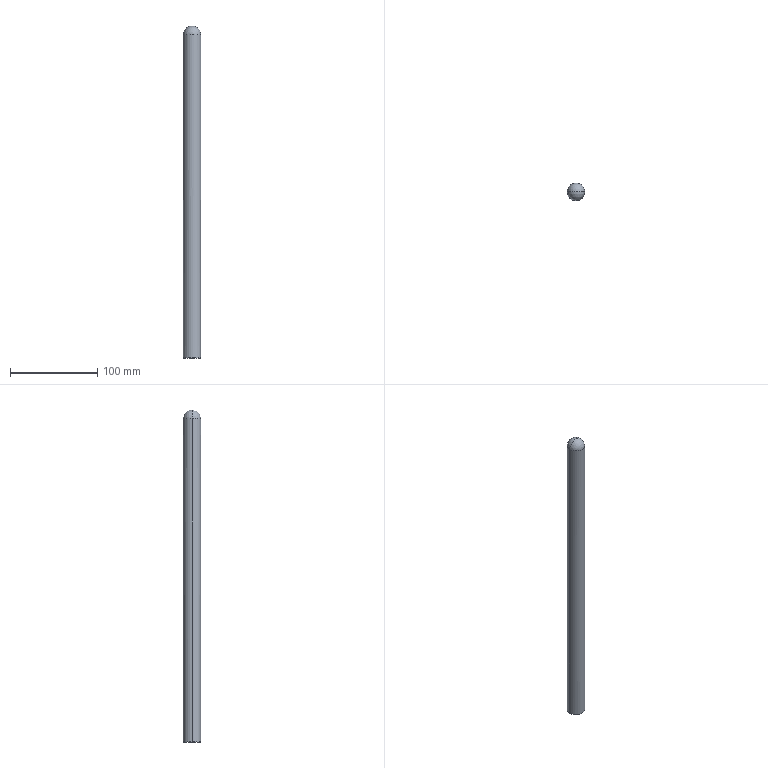Component | SolidWorks | 002MaterialPickingModuleB-1_J-003-2 | 1 solid | 11 faces | box 20 x 20 x 380 mm | volume 117584 mm3 | cone 4 | cylinder 4 | sphere 2 | plane 1 | commonest cylinder face diameters 6.8 x2 20 x2 | material 45
build123d program:
from build123d import *

# Parameters (mm, degrees)
SKETCH1_R             = 10
BOSS_EXTRUDE1_DEPTH   = 380
M8_TAPPED_HOLE1_D     = 6.8
M8_TAPPED_HOLE1_DEPTH = 19.75
M8_TAPPED_HOLE1_TIP   = 2.043
FILLET1_R             = 10
CHAMFER1_SIZE         = 0.5


with BuildPart() as part:
    # Sketch1 → Boss-Extrude1 (new body)
    with BuildSketch(Plane.XY):
        Circle(SKETCH1_R)
    extrude(amount=BOSS_EXTRUDE1_DEPTH)

    # M8 Tapped Hole1
    with Locations(Plane(origin=(0, 0, 0), x_dir=(-1, 0, 0), z_dir=(0, 0, -1))):
        with Locations((0, 0)):
            Hole(M8_TAPPED_HOLE1_D / 2, depth=M8_TAPPED_HOLE1_DEPTH)
            with Locations((0, 0, -(M8_TAPPED_HOLE1_DEPTH + M8_TAPPED_HOLE1_TIP / 2))):  # 118° drill point
                Cone(0, M8_TAPPED_HOLE1_D / 2, M8_TAPPED_HOLE1_TIP, mode=Mode.SUBTRACT)

    # Fillet1
    fillet1_edges = [part.edges().sort_by_distance(p)[0] for p in [
        (-10, 0, 380),
    ]]
    fillet(fillet1_edges, radius=FILLET1_R)

    # Chamfer1
    chamfer1_edges = [part.edges().sort_by_distance(p)[0] for p in [
        (-10, 0, 0),
    ]]
    chamfer(chamfer1_edges, length=CHAMFER1_SIZE)


solid = part.part

# Placed as in the assembly
solid = solid.moved(Location((70.325, 123.019, 113.231), (0, 0, 0)))
STEP:
#1=CARTESIAN_POINT('',(2.395,4.843,4.458));
#2=VERTEX_POINT('',#1);
#3=CARTESIAN_POINT('',(3.143,4.843,4.458));
#4=VERTEX_POINT('',#3);
#5=CARTESIAN_POINT('',(2.769,4.843,4.458));
#6=DIRECTION('',(0.,0.,-1.));
#7=DIRECTION('',(1.,0.,0.));
#8=AXIS2_PLACEMENT_3D('',#5,#6,#7);
#9=CIRCLE('',#8,0.374);
#10=EDGE_CURVE('',#2,#4,#9,.T.);
#11=ORIENTED_EDGE('',*,*,#10,.F.);
#12=CARTESIAN_POINT('',(2.375,4.843,4.478));
#13=VERTEX_POINT('',#12);
#14=CARTESIAN_POINT('',(2.375,4.843,4.478));
#15=DIRECTION('',(-0.7071,0.,0.7071));
#16=VECTOR('',#15,39.37);
#17=LINE('',#14,#16);
#18=EDGE_CURVE('',#2,#13,#17,.T.);
#19=ORIENTED_EDGE('',*,*,#18,.T.);
#20=CARTESIAN_POINT('',(3.162,4.843,4.478));
#21=VERTEX_POINT('',#20);
#22=CARTESIAN_POINT('',(2.769,4.843,4.478));
#23=DIRECTION('',(0.,0.,1.));
#24=DIRECTION('',(1.,0.,0.));
#25=AXIS2_PLACEMENT_3D('',#22,#23,#24);
#26=CIRCLE('',#25,0.3937);
#27=EDGE_CURVE('',#21,#13,#26,.T.);
#28=ORIENTED_EDGE('',*,*,#27,.F.);
#29=CARTESIAN_POINT('',(3.162,4.843,4.478));
#30=DIRECTION('',(0.7071,0.,0.7071));
#31=VECTOR('',#30,39.37);
#32=LINE('',#29,#31);
#33=EDGE_CURVE('',#4,#21,#32,.T.);
#34=ORIENTED_EDGE('',*,*,#33,.F.);
#35=EDGE_LOOP('',(#11,#19,#28,#34));
#36=FACE_OUTER_BOUND('',#35,.T.);
#37=CARTESIAN_POINT('',(2.769,4.843,4.478));
#38=DIRECTION('',(0.,0.,1.));
#39=DIRECTION('',(1.,0.,0.));
#40=AXIS2_PLACEMENT_3D('',#37,#38,#39);
#41=CONICAL_SURFACE('',#40,0.3937,0.7854);
#42=ADVANCED_FACE('',(#36),#41,.T.);
#43=CARTESIAN_POINT('',(2.375,4.843,19.025));
#44=VERTEX_POINT('',#43);
#45=CARTESIAN_POINT('',(3.162,4.843,19.025));
#46=VERTEX_POINT('',#45);
#47=CARTESIAN_POINT('',(2.769,4.843,19.025));
#48=DIRECTION('',(0.,0.,-1.));
#49=DIRECTION('',(-1.,0.,0.));
#50=AXIS2_PLACEMENT_3D('',#47,#48,#49);
#51=CIRCLE('',#50,0.3937);
#52=EDGE_CURVE('',#44,#46,#51,.T.);
#53=ORIENTED_EDGE('',*,*,#52,.F.);
#54=CARTESIAN_POINT('',(2.769,4.843,19.419));
#55=VERTEX_POINT('',#54);
#56=CARTESIAN_POINT('',(2.769,4.843,19.025));
#57=DIRECTION('',(0.,1.,0.));
#58=DIRECTION('',(-1.,0.,0.));
#59=AXIS2_PLACEMENT_3D('',#56,#57,#58);
#60=CIRCLE('',#59,0.3937);
#61=EDGE_CURVE('',#44,#55,#60,.T.);
#62=ORIENTED_EDGE('',*,*,#61,.T.);
#63=CARTESIAN_POINT('',(2.769,4.843,19.025));
#64=DIRECTION('',(0.,-1.,0.));
#65=DIRECTION('',(0.,0.,-1.));
#66=AXIS2_PLACEMENT_3D('',#63,#64,#65);
#67=CIRCLE('',#66,0.3937);
#68=EDGE_CURVE('',#46,#55,#67,.T.);
#69=ORIENTED_EDGE('',*,*,#68,.F.);
#70=EDGE_LOOP('',(#53,#62,#69));
#71=FACE_OUTER_BOUND('',#70,.T.);
#72=CARTESIAN_POINT('',(2.769,4.843,19.025));
#73=DIRECTION('',(0.,1.,0.));
#74=DIRECTION('',(1.,0.,0.));
#75=AXIS2_PLACEMENT_3D('',#72,#73,#74);
#76=SPHERICAL_SURFACE('',#75,0.3937);
#77=ADVANCED_FACE('',(#71),#76,.T.);
#78=CARTESIAN_POINT('',(2.903,4.843,5.235));
#79=VERTEX_POINT('',#78);
#80=CARTESIAN_POINT('',(2.635,4.843,5.235));
#81=VERTEX_POINT('',#80);
#82=CARTESIAN_POINT('',(2.769,4.843,5.235));
#83=DIRECTION('',(0.,0.,-1.));
#84=DIRECTION('',(-1.,0.,0.));
#85=AXIS2_PLACEMENT_3D('',#82,#83,#84);
#86=CIRCLE('',#85,0.1339);
#87=EDGE_CURVE('',#79,#81,#86,.T.);
#88=ORIENTED_EDGE('',*,*,#87,.F.);
#89=CARTESIAN_POINT('',(2.903,4.843,4.458));
#90=VERTEX_POINT('',#89);
#91=CARTESIAN_POINT('',(2.903,4.843,4.458));
#92=DIRECTION('',(0.,0.,-1.));
#93=VECTOR('',#92,39.37);
#94=LINE('',#91,#93);
#95=EDGE_CURVE('',#79,#90,#94,.T.);
#96=ORIENTED_EDGE('',*,*,#95,.T.);
#97=CARTESIAN_POINT('',(2.635,4.843,4.458));
#98=VERTEX_POINT('',#97);
#99=CARTESIAN_POINT('',(2.769,4.843,4.458));
#100=DIRECTION('',(0.,0.,-1.));
#101=DIRECTION('',(-1.,0.,0.));
#102=AXIS2_PLACEMENT_3D('',#99,#100,#101);
#103=CIRCLE('',#102,0.1339);
#104=EDGE_CURVE('',#90,#98,#103,.T.);
#105=ORIENTED_EDGE('',*,*,#104,.T.);
#106=CARTESIAN_POINT('',(2.635,4.843,4.458));
#107=DIRECTION('',(0.,0.,-1.));
#108=VECTOR('',#107,39.37);
#109=LINE('',#106,#108);
#110=EDGE_CURVE('',#81,#98,#109,.T.);
#111=ORIENTED_EDGE('',*,*,#110,.F.);
#112=EDGE_LOOP('',(#88,#96,#105,#111));
#113=FACE_OUTER_BOUND('',#112,.T.);
#114=CARTESIAN_POINT('',(2.769,4.843,4.458));
#115=DIRECTION('',(0.,0.,-1.));
#116=DIRECTION('',(-1.,0.,0.));
#117=AXIS2_PLACEMENT_3D('',#114,#115,#116);
#118=CYLINDRICAL_SURFACE('',#117,0.1339);
#119=ADVANCED_FACE('',(#113),#118,.F.);
#120=CARTESIAN_POINT('',(2.769,4.843,5.316));
#121=VERTEX_POINT('',#120);
#122=CARTESIAN_POINT('',(2.635,4.843,5.235));
#123=DIRECTION('',(-0.8572,0.,-0.515));
#124=VECTOR('',#123,39.37);
#125=LINE('',#122,#124);
#126=EDGE_CURVE('',#121,#81,#125,.T.);
#127=ORIENTED_EDGE('',*,*,#126,.F.);
#128=CARTESIAN_POINT('',(2.903,4.843,5.235));
#129=DIRECTION('',(0.8572,0.,-0.515));
#130=VECTOR('',#129,39.37);
#131=LINE('',#128,#130);
#132=EDGE_CURVE('',#121,#79,#131,.T.);
#133=ORIENTED_EDGE('',*,*,#132,.T.);
#134=ORIENTED_EDGE('',*,*,#87,.T.);
#135=EDGE_LOOP('',(#127,#133,#134));
#136=FACE_OUTER_BOUND('',#135,.T.);
#137=CARTESIAN_POINT('',(2.769,4.843,5.235));
#138=DIRECTION('',(0.,0.,-1.));
#139=DIRECTION('',(-1.,0.,0.));
#140=AXIS2_PLACEMENT_3D('',#137,#138,#139);
#141=CONICAL_SURFACE('',#140,0.1339,1.03);
#142=ADVANCED_FACE('',(#136),#141,.F.);
#143=ORIENTED_EDGE('',*,*,#52,.T.);
#144=CARTESIAN_POINT('',(3.162,4.843,19.419));
#145=DIRECTION('',(0.,0.,-1.));
#146=VECTOR('',#145,39.37);
#147=LINE('',#144,#146);
#148=EDGE_CURVE('',#46,#21,#147,.T.);
#149=ORIENTED_EDGE('',*,*,#148,.T.);
#150=ORIENTED_EDGE('',*,*,#27,.T.);
#151=CARTESIAN_POINT('',(2.375,4.843,19.419));
#152=DIRECTION('',(0.,0.,-1.));
#153=VECTOR('',#152,39.37);
#154=LINE('',#151,#153);
#155=EDGE_CURVE('',#44,#13,#154,.T.);
#156=ORIENTED_EDGE('',*,*,#155,.F.);
#157=EDGE_LOOP('',(#143,#149,#150,#156));
#158=FACE_OUTER_BOUND('',#157,.T.);
#159=CARTESIAN_POINT('',(2.769,4.843,19.419));
#160=DIRECTION('',(0.,0.,-1.));
#161=DIRECTION('',(-1.,0.,0.));
#162=AXIS2_PLACEMENT_3D('',#159,#160,#161);
#163=CYLINDRICAL_SURFACE('',#162,0.3937);
#164=ADVANCED_FACE('',(#158),#163,.T.);
#165=ORIENTED_EDGE('',*,*,#148,.F.);
#166=CARTESIAN_POINT('',(2.769,4.843,19.025));
#167=DIRECTION('',(0.,0.,-1.));
#168=DIRECTION('',(-1.,0.,0.));
#169=AXIS2_PLACEMENT_3D('',#166,#167,#168);
#170=CIRCLE('',#169,0.3937);
#171=EDGE_CURVE('',#46,#44,#170,.T.);
#172=ORIENTED_EDGE('',*,*,#171,.T.);
#173=ORIENTED_EDGE('',*,*,#155,.T.);
#174=CARTESIAN_POINT('',(2.769,4.843,4.478));
#175=DIRECTION('',(0.,0.,1.));
#176=DIRECTION('',(1.,0.,0.));
#177=AXIS2_PLACEMENT_3D('',#174,#175,#176);
#178=CIRCLE('',#177,0.3937);
#179=EDGE_CURVE('',#13,#21,#178,.T.);
#180=ORIENTED_EDGE('',*,*,#179,.T.);
#181=EDGE_LOOP('',(#165,#172,#173,#180));
#182=FACE_OUTER_BOUND('',#181,.T.);
#183=CARTESIAN_POINT('',(2.769,4.843,19.419));
#184=DIRECTION('',(0.,0.,-1.));
#185=DIRECTION('',(-1.,0.,0.));
#186=AXIS2_PLACEMENT_3D('',#183,#184,#185);
#187=CYLINDRICAL_SURFACE('',#186,0.3937);
#188=ADVANCED_FACE('',(#182),#187,.T.);
#189=CARTESIAN_POINT('',(2.769,4.843,4.458));
#190=DIRECTION('',(0.,0.,-1.));
#191=DIRECTION('',(1.,0.,0.));
#192=AXIS2_PLACEMENT_3D('',#189,#190,#191);
#193=CIRCLE('',#192,0.374);
#194=EDGE_CURVE('',#4,#2,#193,.T.);
#195=ORIENTED_EDGE('',*,*,#194,.T.);
#196=ORIENTED_EDGE('',*,*,#10,.T.);
#197=EDGE_LOOP('',(#195,#196));
#198=FACE_OUTER_BOUND('',#197,.T.);
#199=CARTESIAN_POINT('',(2.769,4.843,4.458));
#200=DIRECTION('',(0.,0.,-1.));
#201=DIRECTION('',(-1.,0.,0.));
#202=AXIS2_PLACEMENT_3D('',#199,#200,#201);
#203=CIRCLE('',#202,0.1339);
#204=EDGE_CURVE('',#98,#90,#203,.T.);
#205=ORIENTED_EDGE('',*,*,#204,.F.);
#206=ORIENTED_EDGE('',*,*,#104,.F.);
#207=EDGE_LOOP('',(#205,#206));
#208=FACE_BOUND('',#207,.T.);
#209=CARTESIAN_POINT('',(2.769,4.843,4.458));
#210=DIRECTION('',(0.,0.,1.));
#211=DIRECTION('',(1.,0.,0.));
#212=AXIS2_PLACEMENT_3D('',#209,#210,#211);
#213=PLANE('',#212);
#214=ADVANCED_FACE('',(#198,#208),#213,.F.);
#215=ORIENTED_EDGE('',*,*,#132,.F.);
#216=ORIENTED_EDGE('',*,*,#126,.T.);
#217=CARTESIAN_POINT('',(2.769,4.843,5.235));
#218=DIRECTION('',(0.,0.,-1.));
#219=DIRECTION('',(-1.,0.,0.));
#220=AXIS2_PLACEMENT_3D('',#217,#218,#219);
#221=CIRCLE('',#220,0.1339);
#222=EDGE_CURVE('',#81,#79,#221,.T.);
#223=ORIENTED_EDGE('',*,*,#222,.T.);
#224=EDGE_LOOP('',(#215,#216,#223));
#225=FACE_OUTER_BOUND('',#224,.T.);
#226=CARTESIAN_POINT('',(2.769,4.843,5.235));
#227=DIRECTION('',(0.,0.,-1.));
#228=DIRECTION('',(-1.,0.,0.));
#229=AXIS2_PLACEMENT_3D('',#226,#227,#228);
#230=CONICAL_SURFACE('',#229,0.1339,1.03);
#231=ADVANCED_FACE('',(#225),#230,.F.);
#232=ORIENTED_EDGE('',*,*,#95,.F.);
#233=ORIENTED_EDGE('',*,*,#222,.F.);
#234=ORIENTED_EDGE('',*,*,#110,.T.);
#235=ORIENTED_EDGE('',*,*,#204,.T.);
#236=EDGE_LOOP('',(#232,#233,#234,#235));
#237=FACE_OUTER_BOUND('',#236,.T.);
#238=CARTESIAN_POINT('',(2.769,4.843,4.458));
#239=DIRECTION('',(0.,0.,-1.));
#240=DIRECTION('',(-1.,0.,0.));
#241=AXIS2_PLACEMENT_3D('',#238,#239,#240);
#242=CYLINDRICAL_SURFACE('',#241,0.1339);
#243=ADVANCED_FACE('',(#237),#242,.F.);
#244=ORIENTED_EDGE('',*,*,#61,.F.);
#245=ORIENTED_EDGE('',*,*,#171,.F.);
#246=ORIENTED_EDGE('',*,*,#68,.T.);
#247=EDGE_LOOP('',(#244,#245,#246));
#248=FACE_OUTER_BOUND('',#247,.T.);
#249=CARTESIAN_POINT('',(2.769,4.843,19.025));
#250=DIRECTION('',(0.,1.,0.));
#251=DIRECTION('',(1.,0.,0.));
#252=AXIS2_PLACEMENT_3D('',#249,#250,#251);
#253=SPHERICAL_SURFACE('',#252,0.3937);
#254=ADVANCED_FACE('',(#248),#253,.T.);
#255=ORIENTED_EDGE('',*,*,#18,.F.);
#256=ORIENTED_EDGE('',*,*,#194,.F.);
#257=ORIENTED_EDGE('',*,*,#33,.T.);
#258=ORIENTED_EDGE('',*,*,#179,.F.);
#259=EDGE_LOOP('',(#255,#256,#257,#258));
#260=FACE_OUTER_BOUND('',#259,.T.);
#261=CARTESIAN_POINT('',(2.769,4.843,4.478));
#262=DIRECTION('',(0.,0.,1.));
#263=DIRECTION('',(1.,0.,0.));
#264=AXIS2_PLACEMENT_3D('',#261,#262,#263);
#265=CONICAL_SURFACE('',#264,0.3937,0.7854);
#266=ADVANCED_FACE('',(#260),#265,.T.);
#267=CLOSED_SHELL('',(#42,#77,#119,#142,#164,#188,#214,#231,#243,#254,#266));
#268=MANIFOLD_SOLID_BREP('',#267);
#269=CARTESIAN_POINT('',(0.,0.,0.));
#270=DIRECTION('',(0.,0.,1.));
#271=DIRECTION('',(1.,0.,0.));
#272=AXIS2_PLACEMENT_3D('',#269,#270,#271);
#273=(LENGTH_UNIT()NAMED_UNIT(*)SI_UNIT($,.METRE.));
#274=LENGTH_MEASURE_WITH_UNIT(LENGTH_MEASURE(0.0254),#273);
#275=DIMENSIONAL_EXPONENTS(1.,0.,0.,0.,0.,0.,0.);
#276=(CONVERSION_BASED_UNIT('',#274)LENGTH_UNIT()NAMED_UNIT(#275));
#277=UNCERTAINTY_MEASURE_WITH_UNIT(LENGTH_MEASURE(0.00001),#276,'','');
#278=(NAMED_UNIT(*)PLANE_ANGLE_UNIT()SI_UNIT($,.RADIAN.));
#279=(NAMED_UNIT(*)SI_UNIT($,.STERADIAN.)SOLID_ANGLE_UNIT());
#280=(GEOMETRIC_REPRESENTATION_CONTEXT(3)GLOBAL_UNCERTAINTY_ASSIGNED_CONTEXT((#277))GLOBAL_UNIT_ASSIGNED_CONTEXT((#276,#278,#279))REPRESENTATION_CONTEXT('',''));
#281=ADVANCED_BREP_SHAPE_REPRESENTATION('',(#268,#272),#280);
#282=COLOUR_RGB('',0.7922,0.8196,0.9333);
#283=FILL_AREA_STYLE_COLOUR('',#282);
#284=FILL_AREA_STYLE('',(#283));
#285=SURFACE_STYLE_FILL_AREA(#284);
#286=SURFACE_SIDE_STYLE('',(#285));
#287=SURFACE_STYLE_USAGE(.BOTH.,#286);
#288=PRESENTATION_STYLE_ASSIGNMENT((#287));
#289=STYLED_ITEM('',(#288),#268);
#290=(LENGTH_UNIT()NAMED_UNIT(*)SI_UNIT($,.METRE.));
#291=LENGTH_MEASURE_WITH_UNIT(LENGTH_MEASURE(0.0254),#290);
#292=DIMENSIONAL_EXPONENTS(1.,0.,0.,0.,0.,0.,0.);
#293=(CONVERSION_BASED_UNIT('',#291)LENGTH_UNIT()NAMED_UNIT(#292));
#294=UNCERTAINTY_MEASURE_WITH_UNIT(LENGTH_MEASURE(0.00001),#293,'','');
#295=(NAMED_UNIT(*)PLANE_ANGLE_UNIT()SI_UNIT($,.RADIAN.));
#296=(NAMED_UNIT(*)SI_UNIT($,.STERADIAN.)SOLID_ANGLE_UNIT());
#297=(GEOMETRIC_REPRESENTATION_CONTEXT(3)GLOBAL_UNCERTAINTY_ASSIGNED_CONTEXT((#294))GLOBAL_UNIT_ASSIGNED_CONTEXT((#293,#295,#296))REPRESENTATION_CONTEXT('',''));
#298=MECHANICAL_DESIGN_GEOMETRIC_PRESENTATION_REPRESENTATION('',(#289),#297);
#299=PRESENTATION_LAYER_ASSIGNMENT('','',(#289));